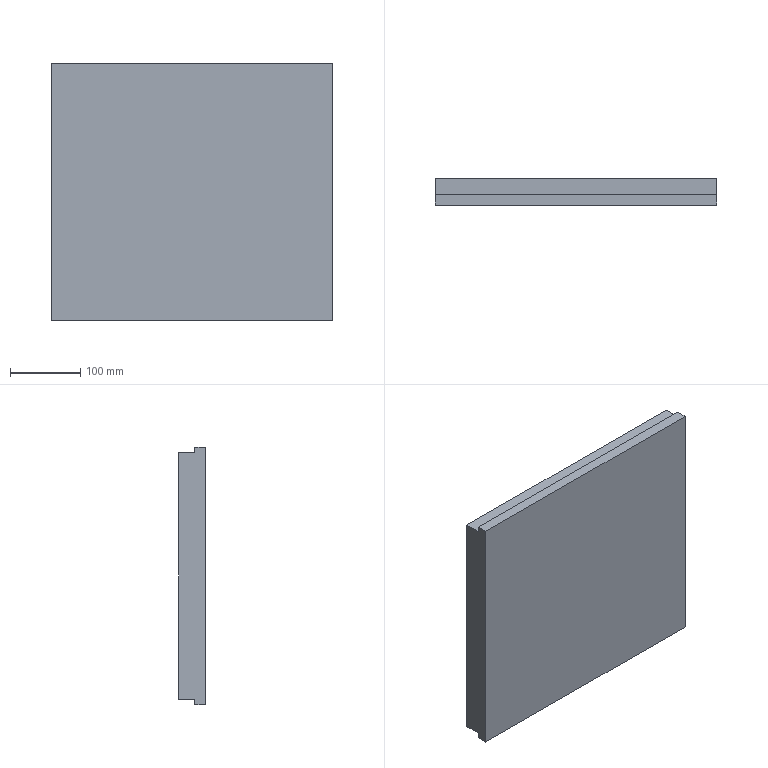Component | SolidWorks | NewDieSet-1_LowerDieSetAssembly-1_MoldPlate-1 | 1 solid | 10 faces | box 400 x 38 x 366 mm | volume 5416000 mm3 | plane 10
build123d program:
from build123d import *

# Parameters (mm, degrees)
SKETCH1_W           = 400
SKETCH1_H           = 366
BOSS_EXTRUDE1_DEPTH = 38
SKETCH8_W           = 8
SKETCH8_H           = 23
CUT_EXTRUDE5_DEPTH  = 544.507


with BuildPart() as part:
    # Sketch1 → Boss-Extrude1 (new body)
    with BuildSketch(Plane(origin=(0, 0, 0), x_dir=(1, 0, 0), z_dir=(0, 1, 0))):
        with Locations((200, 183)):
            Rectangle(SKETCH1_W, SKETCH1_H)
    extrude(amount=BOSS_EXTRUDE1_DEPTH)

    # Sketch8 → Cut-Extrude5 (cut, through all)
    with BuildSketch(Plane(origin=(400, 0, 0), x_dir=(0, 0, -1), z_dir=(1, 0, 0))):
        with Locations((362, 11.5)):
            Rectangle(SKETCH8_W, SKETCH8_H)
        with Locations((4, 11.5)):
            Rectangle(SKETCH8_W, SKETCH8_H)
    extrude(amount=-CUT_EXTRUDE5_DEPTH, mode=Mode.SUBTRACT)


solid = part.part

# Placed as in the assembly
solid = solid.moved(Location((-256.746, 43.927, 170), (180, 0, 0)))
STEP:
#1=CARTESIAN_POINT('',(5.64,1.729,20.787));
#2=VERTEX_POINT('',#1);
#3=CARTESIAN_POINT('',(5.64,0.8239,20.787));
#4=VERTEX_POINT('',#3);
#5=CARTESIAN_POINT('',(5.64,1.729,20.787));
#6=DIRECTION('',(0.,-1.,0.));
#7=VECTOR('',#6,39.37);
#8=LINE('',#5,#7);
#9=EDGE_CURVE('',#2,#4,#8,.T.);
#10=ORIENTED_EDGE('',*,*,#9,.T.);
#11=CARTESIAN_POINT('',(5.64,0.8239,21.102));
#12=VERTEX_POINT('',#11);
#13=CARTESIAN_POINT('',(5.64,0.8239,21.102));
#14=DIRECTION('',(0.,0.,1.));
#15=VECTOR('',#14,39.37);
#16=LINE('',#13,#15);
#17=EDGE_CURVE('',#4,#12,#16,.T.);
#18=ORIENTED_EDGE('',*,*,#17,.T.);
#19=CARTESIAN_POINT('',(5.64,0.2333,21.102));
#20=VERTEX_POINT('',#19);
#21=CARTESIAN_POINT('',(5.64,0.2333,21.102));
#22=DIRECTION('',(0.,1.,0.));
#23=VECTOR('',#22,39.37);
#24=LINE('',#21,#23);
#25=EDGE_CURVE('',#20,#12,#24,.T.);
#26=ORIENTED_EDGE('',*,*,#25,.F.);
#27=CARTESIAN_POINT('',(5.64,0.2333,6.693));
#28=VERTEX_POINT('',#27);
#29=CARTESIAN_POINT('',(5.64,0.2333,21.102));
#30=DIRECTION('',(0.,0.,1.));
#31=VECTOR('',#30,39.37);
#32=LINE('',#29,#31);
#33=EDGE_CURVE('',#28,#20,#32,.T.);
#34=ORIENTED_EDGE('',*,*,#33,.F.);
#35=CARTESIAN_POINT('',(5.64,0.8239,6.693));
#36=VERTEX_POINT('',#35);
#37=CARTESIAN_POINT('',(5.64,0.2333,6.693));
#38=DIRECTION('',(0.,1.,0.));
#39=VECTOR('',#38,39.37);
#40=LINE('',#37,#39);
#41=EDGE_CURVE('',#28,#36,#40,.T.);
#42=ORIENTED_EDGE('',*,*,#41,.T.);
#43=CARTESIAN_POINT('',(5.64,0.8239,7.008));
#44=VERTEX_POINT('',#43);
#45=CARTESIAN_POINT('',(5.64,0.8239,6.693));
#46=DIRECTION('',(0.,0.,1.));
#47=VECTOR('',#46,39.37);
#48=LINE('',#45,#47);
#49=EDGE_CURVE('',#36,#44,#48,.T.);
#50=ORIENTED_EDGE('',*,*,#49,.T.);
#51=CARTESIAN_POINT('',(5.64,1.729,7.008));
#52=VERTEX_POINT('',#51);
#53=CARTESIAN_POINT('',(5.64,1.729,7.008));
#54=DIRECTION('',(0.,1.,0.));
#55=VECTOR('',#54,39.37);
#56=LINE('',#53,#55);
#57=EDGE_CURVE('',#44,#52,#56,.T.);
#58=ORIENTED_EDGE('',*,*,#57,.T.);
#59=CARTESIAN_POINT('',(5.64,1.729,21.102));
#60=DIRECTION('',(0.,0.,1.));
#61=VECTOR('',#60,39.37);
#62=LINE('',#59,#61);
#63=EDGE_CURVE('',#52,#2,#62,.T.);
#64=ORIENTED_EDGE('',*,*,#63,.T.);
#65=EDGE_LOOP('',(#10,#18,#26,#34,#42,#50,#58,#64));
#66=FACE_OUTER_BOUND('',#65,.T.);
#67=CARTESIAN_POINT('',(5.64,0.2333,21.102));
#68=DIRECTION('',(-1.,0.,0.));
#69=DIRECTION('',(-0.,0.,-1.));
#70=AXIS2_PLACEMENT_3D('',#67,#68,#69);
#71=PLANE('',#70);
#72=ADVANCED_FACE('',(#66),#71,.F.);
#73=ORIENTED_EDGE('',*,*,#25,.T.);
#74=CARTESIAN_POINT('',(-10.108,0.8239,21.102));
#75=VERTEX_POINT('',#74);
#76=CARTESIAN_POINT('',(5.64,0.8239,21.102));
#77=DIRECTION('',(-1.,0.,0.));
#78=VECTOR('',#77,39.37);
#79=LINE('',#76,#78);
#80=EDGE_CURVE('',#12,#75,#79,.T.);
#81=ORIENTED_EDGE('',*,*,#80,.T.);
#82=CARTESIAN_POINT('',(-10.108,0.2333,21.102));
#83=VERTEX_POINT('',#82);
#84=CARTESIAN_POINT('',(-10.108,0.2333,21.102));
#85=DIRECTION('',(0.,1.,0.));
#86=VECTOR('',#85,39.37);
#87=LINE('',#84,#86);
#88=EDGE_CURVE('',#83,#75,#87,.T.);
#89=ORIENTED_EDGE('',*,*,#88,.F.);
#90=CARTESIAN_POINT('',(5.64,0.2333,21.102));
#91=DIRECTION('',(-1.,0.,0.));
#92=VECTOR('',#91,39.37);
#93=LINE('',#90,#92);
#94=EDGE_CURVE('',#20,#83,#93,.T.);
#95=ORIENTED_EDGE('',*,*,#94,.F.);
#96=EDGE_LOOP('',(#73,#81,#89,#95));
#97=FACE_OUTER_BOUND('',#96,.T.);
#98=CARTESIAN_POINT('',(5.64,0.2333,21.102));
#99=DIRECTION('',(-0.,0.,-1.));
#100=DIRECTION('',(1.,0.,-0.));
#101=AXIS2_PLACEMENT_3D('',#98,#99,#100);
#102=PLANE('',#101);
#103=ADVANCED_FACE('',(#97),#102,.F.);
#104=ORIENTED_EDGE('',*,*,#88,.T.);
#105=CARTESIAN_POINT('',(-10.108,0.8239,20.787));
#106=VERTEX_POINT('',#105);
#107=CARTESIAN_POINT('',(-10.108,0.8239,21.102));
#108=DIRECTION('',(0.,0.,1.));
#109=VECTOR('',#108,39.37);
#110=LINE('',#107,#109);
#111=EDGE_CURVE('',#106,#75,#110,.T.);
#112=ORIENTED_EDGE('',*,*,#111,.F.);
#113=CARTESIAN_POINT('',(-10.108,1.729,20.787));
#114=VERTEX_POINT('',#113);
#115=CARTESIAN_POINT('',(-10.108,1.729,20.787));
#116=DIRECTION('',(0.,-1.,0.));
#117=VECTOR('',#116,39.37);
#118=LINE('',#115,#117);
#119=EDGE_CURVE('',#114,#106,#118,.T.);
#120=ORIENTED_EDGE('',*,*,#119,.F.);
#121=CARTESIAN_POINT('',(-10.108,1.729,7.008));
#122=VERTEX_POINT('',#121);
#123=CARTESIAN_POINT('',(-10.108,1.729,21.102));
#124=DIRECTION('',(-0.,0.,-1.));
#125=VECTOR('',#124,39.37);
#126=LINE('',#123,#125);
#127=EDGE_CURVE('',#114,#122,#126,.T.);
#128=ORIENTED_EDGE('',*,*,#127,.T.);
#129=CARTESIAN_POINT('',(-10.108,0.8239,7.008));
#130=VERTEX_POINT('',#129);
#131=CARTESIAN_POINT('',(-10.108,1.729,7.008));
#132=DIRECTION('',(0.,1.,0.));
#133=VECTOR('',#132,39.37);
#134=LINE('',#131,#133);
#135=EDGE_CURVE('',#130,#122,#134,.T.);
#136=ORIENTED_EDGE('',*,*,#135,.F.);
#137=CARTESIAN_POINT('',(-10.108,0.8239,6.693));
#138=VERTEX_POINT('',#137);
#139=CARTESIAN_POINT('',(-10.108,0.8239,6.693));
#140=DIRECTION('',(0.,0.,1.));
#141=VECTOR('',#140,39.37);
#142=LINE('',#139,#141);
#143=EDGE_CURVE('',#138,#130,#142,.T.);
#144=ORIENTED_EDGE('',*,*,#143,.F.);
#145=CARTESIAN_POINT('',(-10.108,0.2333,6.693));
#146=VERTEX_POINT('',#145);
#147=CARTESIAN_POINT('',(-10.108,0.2333,6.693));
#148=DIRECTION('',(0.,1.,0.));
#149=VECTOR('',#148,39.37);
#150=LINE('',#147,#149);
#151=EDGE_CURVE('',#146,#138,#150,.T.);
#152=ORIENTED_EDGE('',*,*,#151,.F.);
#153=CARTESIAN_POINT('',(-10.108,0.2333,21.102));
#154=DIRECTION('',(-0.,0.,-1.));
#155=VECTOR('',#154,39.37);
#156=LINE('',#153,#155);
#157=EDGE_CURVE('',#83,#146,#156,.T.);
#158=ORIENTED_EDGE('',*,*,#157,.F.);
#159=EDGE_LOOP('',(#104,#112,#120,#128,#136,#144,#152,#158));
#160=FACE_OUTER_BOUND('',#159,.T.);
#161=CARTESIAN_POINT('',(-10.108,0.2333,21.102));
#162=DIRECTION('',(1.,0.,-0.));
#163=DIRECTION('',(0.,0.,1.));
#164=AXIS2_PLACEMENT_3D('',#161,#162,#163);
#165=PLANE('',#164);
#166=ADVANCED_FACE('',(#160),#165,.F.);
#167=ORIENTED_EDGE('',*,*,#151,.T.);
#168=CARTESIAN_POINT('',(5.64,0.8239,6.693));
#169=DIRECTION('',(-1.,0.,0.));
#170=VECTOR('',#169,39.37);
#171=LINE('',#168,#170);
#172=EDGE_CURVE('',#36,#138,#171,.T.);
#173=ORIENTED_EDGE('',*,*,#172,.F.);
#174=ORIENTED_EDGE('',*,*,#41,.F.);
#175=CARTESIAN_POINT('',(5.64,0.2333,6.693));
#176=DIRECTION('',(1.,0.,-0.));
#177=VECTOR('',#176,39.37);
#178=LINE('',#175,#177);
#179=EDGE_CURVE('',#146,#28,#178,.T.);
#180=ORIENTED_EDGE('',*,*,#179,.F.);
#181=EDGE_LOOP('',(#167,#173,#174,#180));
#182=FACE_OUTER_BOUND('',#181,.T.);
#183=CARTESIAN_POINT('',(5.64,0.2333,6.693));
#184=DIRECTION('',(0.,0.,1.));
#185=DIRECTION('',(-1.,0.,0.));
#186=AXIS2_PLACEMENT_3D('',#183,#184,#185);
#187=PLANE('',#186);
#188=ADVANCED_FACE('',(#182),#187,.F.);
#189=ORIENTED_EDGE('',*,*,#33,.T.);
#190=ORIENTED_EDGE('',*,*,#94,.T.);
#191=ORIENTED_EDGE('',*,*,#157,.T.);
#192=ORIENTED_EDGE('',*,*,#179,.T.);
#193=EDGE_LOOP('',(#189,#190,#191,#192));
#194=FACE_OUTER_BOUND('',#193,.T.);
#195=CARTESIAN_POINT('',(5.64,0.2333,21.102));
#196=DIRECTION('',(0.,1.,0.));
#197=DIRECTION('',(-0.,0.,-1.));
#198=AXIS2_PLACEMENT_3D('',#195,#196,#197);
#199=PLANE('',#198);
#200=ADVANCED_FACE('',(#194),#199,.F.);
#201=CARTESIAN_POINT('',(5.64,1.729,20.787));
#202=DIRECTION('',(-1.,0.,0.));
#203=VECTOR('',#202,39.37);
#204=LINE('',#201,#203);
#205=EDGE_CURVE('',#2,#114,#204,.T.);
#206=ORIENTED_EDGE('',*,*,#205,.F.);
#207=ORIENTED_EDGE('',*,*,#63,.F.);
#208=CARTESIAN_POINT('',(5.64,1.729,7.008));
#209=DIRECTION('',(-1.,0.,0.));
#210=VECTOR('',#209,39.37);
#211=LINE('',#208,#210);
#212=EDGE_CURVE('',#52,#122,#211,.T.);
#213=ORIENTED_EDGE('',*,*,#212,.T.);
#214=ORIENTED_EDGE('',*,*,#127,.F.);
#215=EDGE_LOOP('',(#206,#207,#213,#214));
#216=FACE_OUTER_BOUND('',#215,.T.);
#217=CARTESIAN_POINT('',(5.64,1.729,21.102));
#218=DIRECTION('',(0.,1.,0.));
#219=DIRECTION('',(-0.,0.,-1.));
#220=AXIS2_PLACEMENT_3D('',#217,#218,#219);
#221=PLANE('',#220);
#222=ADVANCED_FACE('',(#216),#221,.T.);
#223=ORIENTED_EDGE('',*,*,#135,.T.);
#224=ORIENTED_EDGE('',*,*,#212,.F.);
#225=ORIENTED_EDGE('',*,*,#57,.F.);
#226=CARTESIAN_POINT('',(5.64,0.8239,7.008));
#227=DIRECTION('',(-1.,0.,0.));
#228=VECTOR('',#227,39.37);
#229=LINE('',#226,#228);
#230=EDGE_CURVE('',#44,#130,#229,.T.);
#231=ORIENTED_EDGE('',*,*,#230,.T.);
#232=EDGE_LOOP('',(#223,#224,#225,#231));
#233=FACE_OUTER_BOUND('',#232,.T.);
#234=CARTESIAN_POINT('',(5.64,1.729,7.008));
#235=DIRECTION('',(0.,0.,1.));
#236=DIRECTION('',(-1.,0.,0.));
#237=AXIS2_PLACEMENT_3D('',#234,#235,#236);
#238=PLANE('',#237);
#239=ADVANCED_FACE('',(#233),#238,.F.);
#240=ORIENTED_EDGE('',*,*,#143,.T.);
#241=ORIENTED_EDGE('',*,*,#230,.F.);
#242=ORIENTED_EDGE('',*,*,#49,.F.);
#243=ORIENTED_EDGE('',*,*,#172,.T.);
#244=EDGE_LOOP('',(#240,#241,#242,#243));
#245=FACE_OUTER_BOUND('',#244,.T.);
#246=CARTESIAN_POINT('',(5.64,0.8239,6.693));
#247=DIRECTION('',(0.,-1.,0.));
#248=DIRECTION('',(0.,0.,1.));
#249=AXIS2_PLACEMENT_3D('',#246,#247,#248);
#250=PLANE('',#249);
#251=ADVANCED_FACE('',(#245),#250,.F.);
#252=ORIENTED_EDGE('',*,*,#111,.T.);
#253=ORIENTED_EDGE('',*,*,#80,.F.);
#254=ORIENTED_EDGE('',*,*,#17,.F.);
#255=CARTESIAN_POINT('',(5.64,0.8239,20.787));
#256=DIRECTION('',(-1.,0.,0.));
#257=VECTOR('',#256,39.37);
#258=LINE('',#255,#257);
#259=EDGE_CURVE('',#4,#106,#258,.T.);
#260=ORIENTED_EDGE('',*,*,#259,.T.);
#261=EDGE_LOOP('',(#252,#253,#254,#260));
#262=FACE_OUTER_BOUND('',#261,.T.);
#263=CARTESIAN_POINT('',(5.64,0.8239,21.102));
#264=DIRECTION('',(0.,-1.,0.));
#265=DIRECTION('',(0.,0.,1.));
#266=AXIS2_PLACEMENT_3D('',#263,#264,#265);
#267=PLANE('',#266);
#268=ADVANCED_FACE('',(#262),#267,.F.);
#269=ORIENTED_EDGE('',*,*,#119,.T.);
#270=ORIENTED_EDGE('',*,*,#259,.F.);
#271=ORIENTED_EDGE('',*,*,#9,.F.);
#272=ORIENTED_EDGE('',*,*,#205,.T.);
#273=EDGE_LOOP('',(#269,#270,#271,#272));
#274=FACE_OUTER_BOUND('',#273,.T.);
#275=CARTESIAN_POINT('',(5.64,1.729,20.787));
#276=DIRECTION('',(-0.,0.,-1.));
#277=DIRECTION('',(1.,0.,-0.));
#278=AXIS2_PLACEMENT_3D('',#275,#276,#277);
#279=PLANE('',#278);
#280=ADVANCED_FACE('',(#274),#279,.F.);
#281=CLOSED_SHELL('',(#72,#103,#166,#188,#200,#222,#239,#251,#268,#280));
#282=MANIFOLD_SOLID_BREP('',#281);
#283=CARTESIAN_POINT('',(0.,0.,0.));
#284=DIRECTION('',(0.,0.,1.));
#285=DIRECTION('',(1.,0.,0.));
#286=AXIS2_PLACEMENT_3D('',#283,#284,#285);
#287=(LENGTH_UNIT()NAMED_UNIT(*)SI_UNIT($,.METRE.));
#288=LENGTH_MEASURE_WITH_UNIT(LENGTH_MEASURE(0.0254),#287);
#289=DIMENSIONAL_EXPONENTS(1.,0.,0.,0.,0.,0.,0.);
#290=(CONVERSION_BASED_UNIT('',#288)LENGTH_UNIT()NAMED_UNIT(#289));
#291=UNCERTAINTY_MEASURE_WITH_UNIT(LENGTH_MEASURE(0.00001),#290,'','');
#292=(NAMED_UNIT(*)PLANE_ANGLE_UNIT()SI_UNIT($,.RADIAN.));
#293=(NAMED_UNIT(*)SI_UNIT($,.STERADIAN.)SOLID_ANGLE_UNIT());
#294=(GEOMETRIC_REPRESENTATION_CONTEXT(3)GLOBAL_UNCERTAINTY_ASSIGNED_CONTEXT((#291))GLOBAL_UNIT_ASSIGNED_CONTEXT((#290,#292,#293))REPRESENTATION_CONTEXT('',''));
#295=ADVANCED_BREP_SHAPE_REPRESENTATION('',(#282,#286),#294);
#296=COLOUR_RGB('',0.7922,0.8196,0.9333);
#297=FILL_AREA_STYLE_COLOUR('',#296);
#298=FILL_AREA_STYLE('',(#297));
#299=SURFACE_STYLE_FILL_AREA(#298);
#300=SURFACE_SIDE_STYLE('',(#299));
#301=SURFACE_STYLE_USAGE(.BOTH.,#300);
#302=PRESENTATION_STYLE_ASSIGNMENT((#301));
#303=STYLED_ITEM('',(#302),#282);
#304=PRESENTATION_LAYER_ASSIGNMENT('','',(#303));
#305=(LENGTH_UNIT()NAMED_UNIT(*)SI_UNIT($,.METRE.));
#306=LENGTH_MEASURE_WITH_UNIT(LENGTH_MEASURE(0.0254),#305);
#307=DIMENSIONAL_EXPONENTS(1.,0.,0.,0.,0.,0.,0.);
#308=(CONVERSION_BASED_UNIT('',#306)LENGTH_UNIT()NAMED_UNIT(#307));
#309=UNCERTAINTY_MEASURE_WITH_UNIT(LENGTH_MEASURE(0.00001),#308,'','');
#310=(NAMED_UNIT(*)PLANE_ANGLE_UNIT()SI_UNIT($,.RADIAN.));
#311=(NAMED_UNIT(*)SI_UNIT($,.STERADIAN.)SOLID_ANGLE_UNIT());
#312=(GEOMETRIC_REPRESENTATION_CONTEXT(3)GLOBAL_UNCERTAINTY_ASSIGNED_CONTEXT((#309))GLOBAL_UNIT_ASSIGNED_CONTEXT((#308,#310,#311))REPRESENTATION_CONTEXT('',''));
#313=MECHANICAL_DESIGN_GEOMETRIC_PRESENTATION_REPRESENTATION('',(#303),#312);